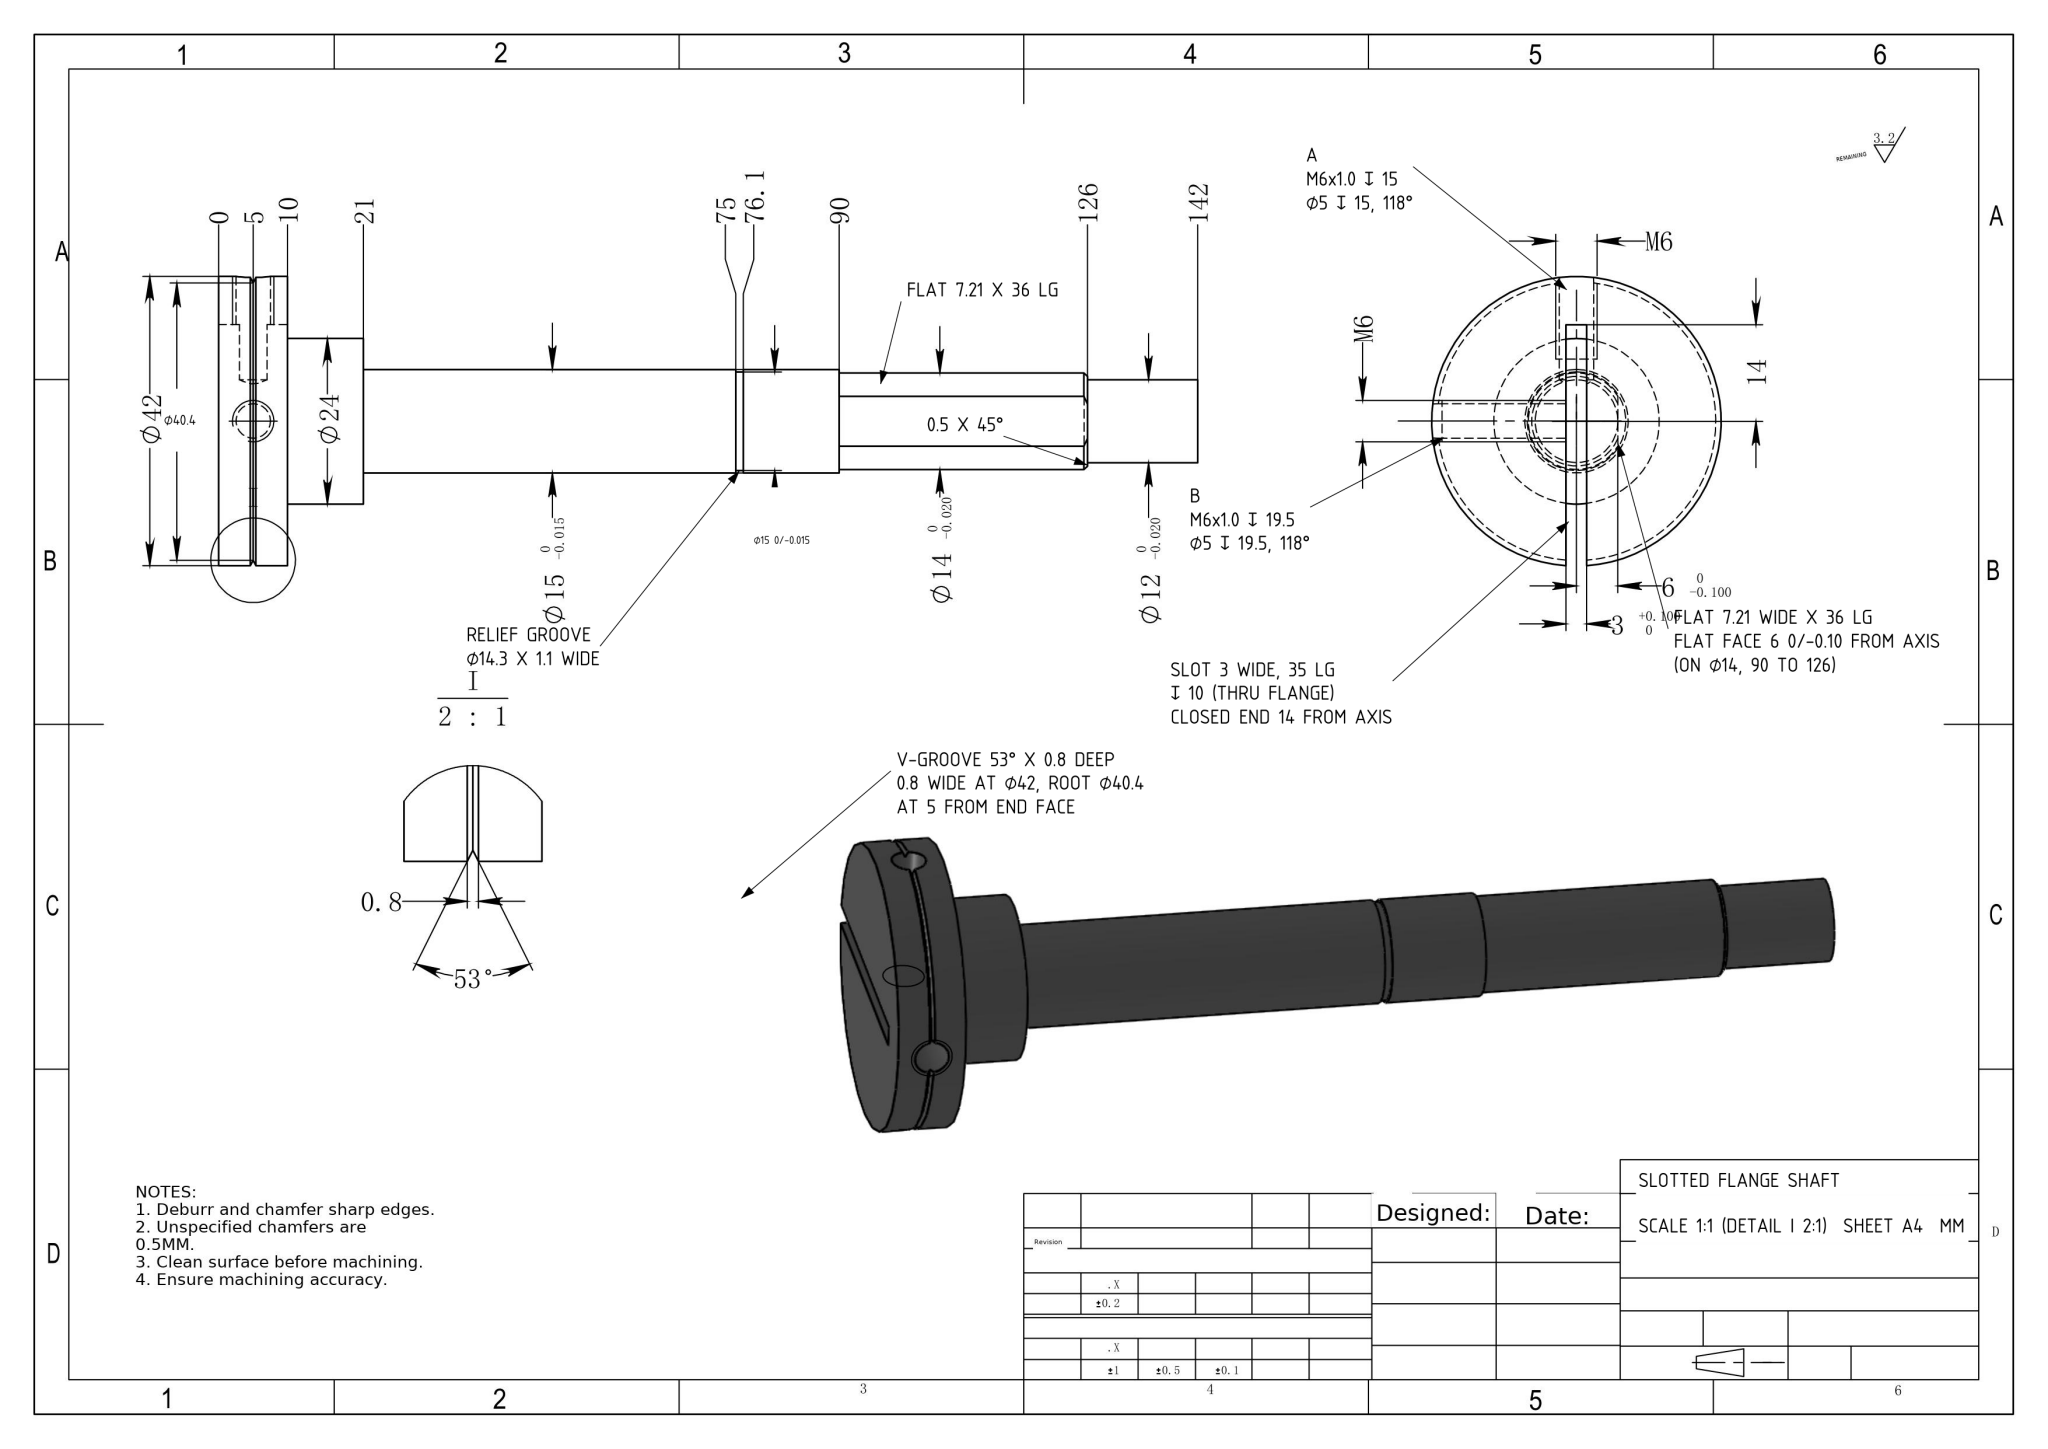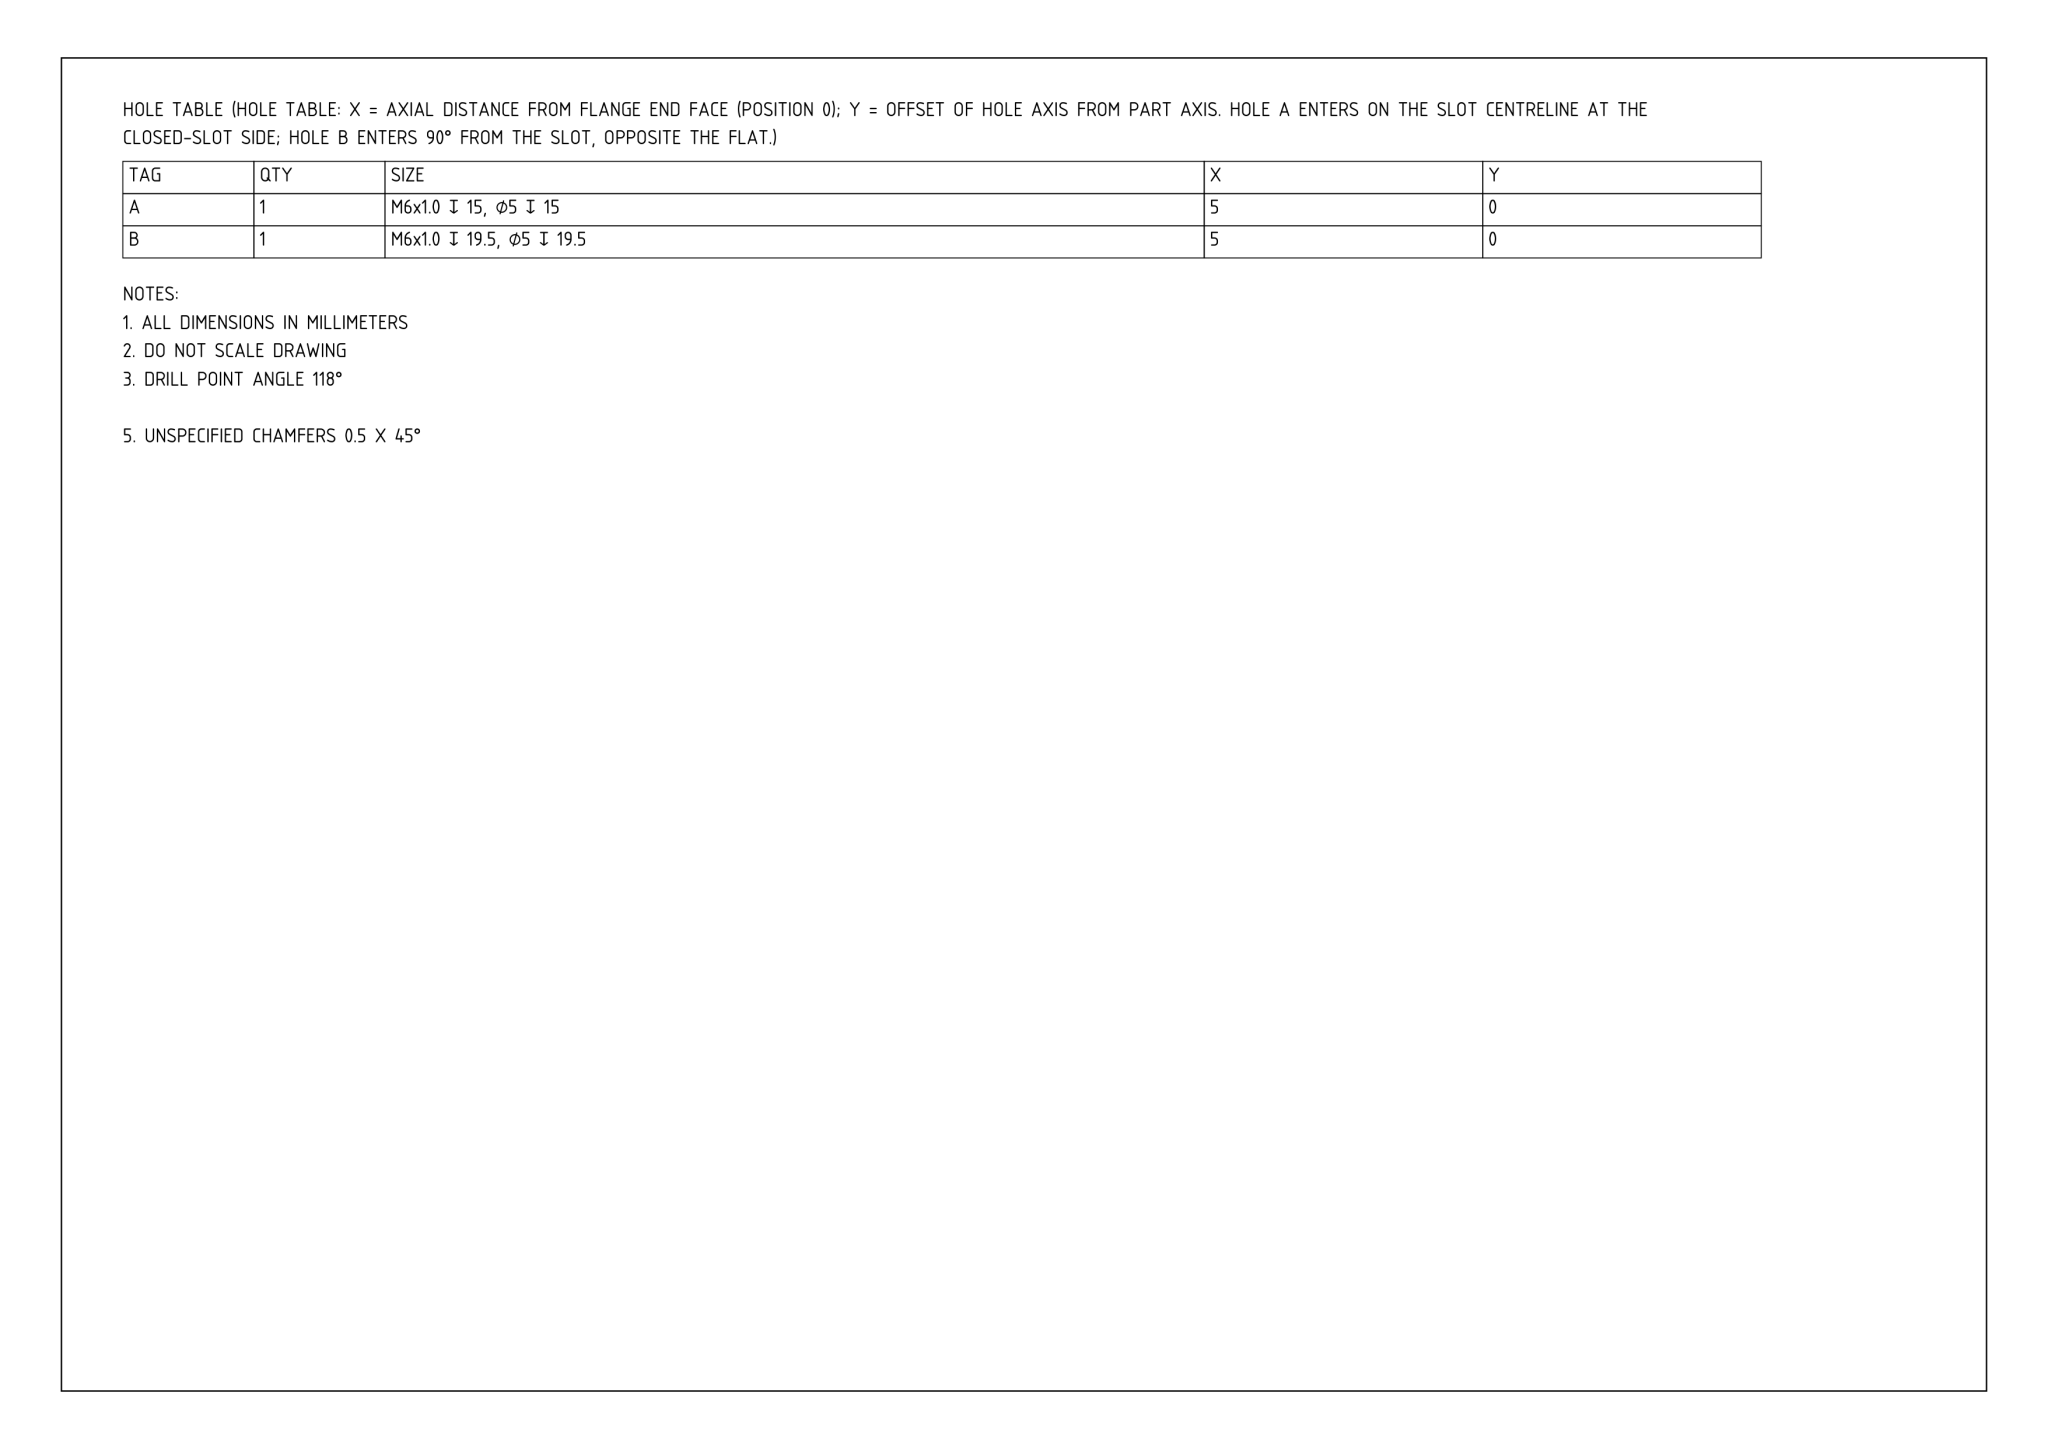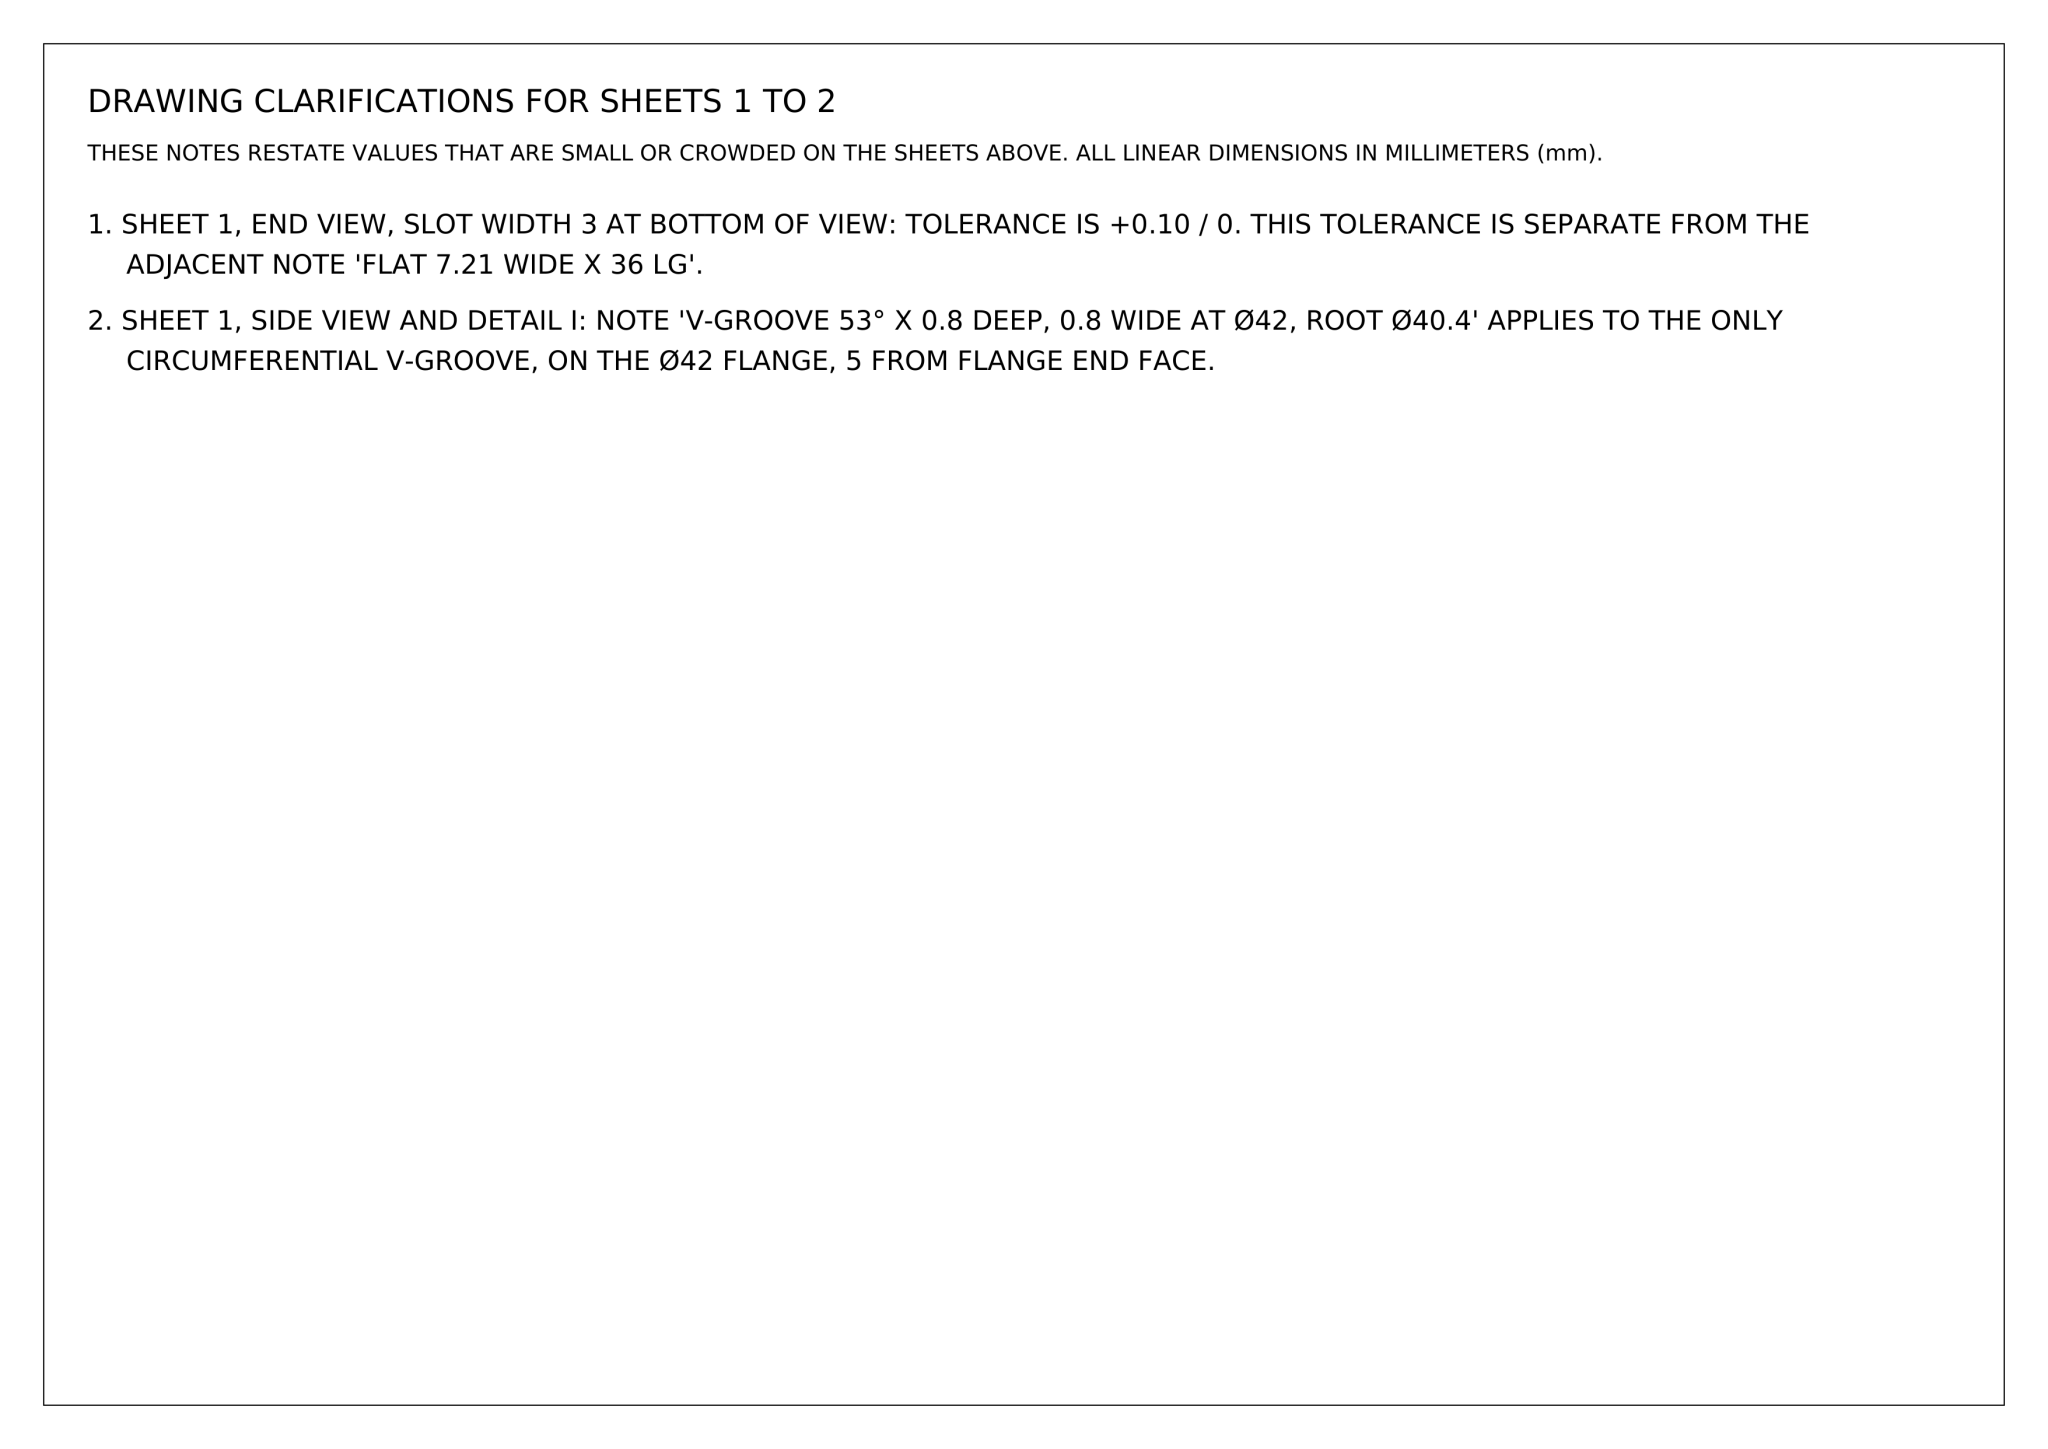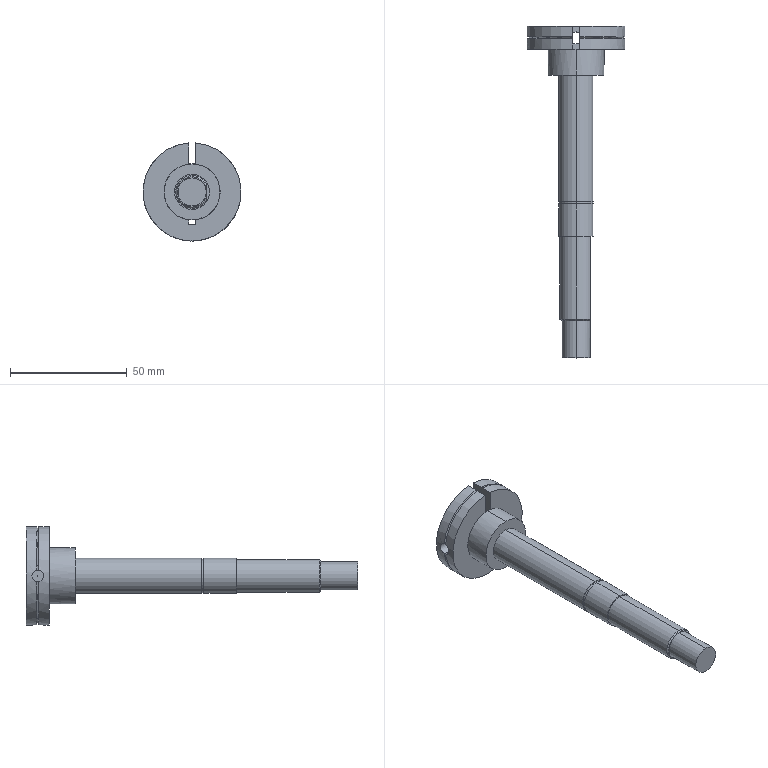Part | NX | mm | 1 solid | 49 faces | box 42 x 142 x 41.95 mm | volume 36526 mm3 | cylinder 21 | cone 14 | plane 14 | commonest cylinder face diameters 5 x4 15 x4 42 x4 14 x3 12 x2 14.3 x2 24 x2